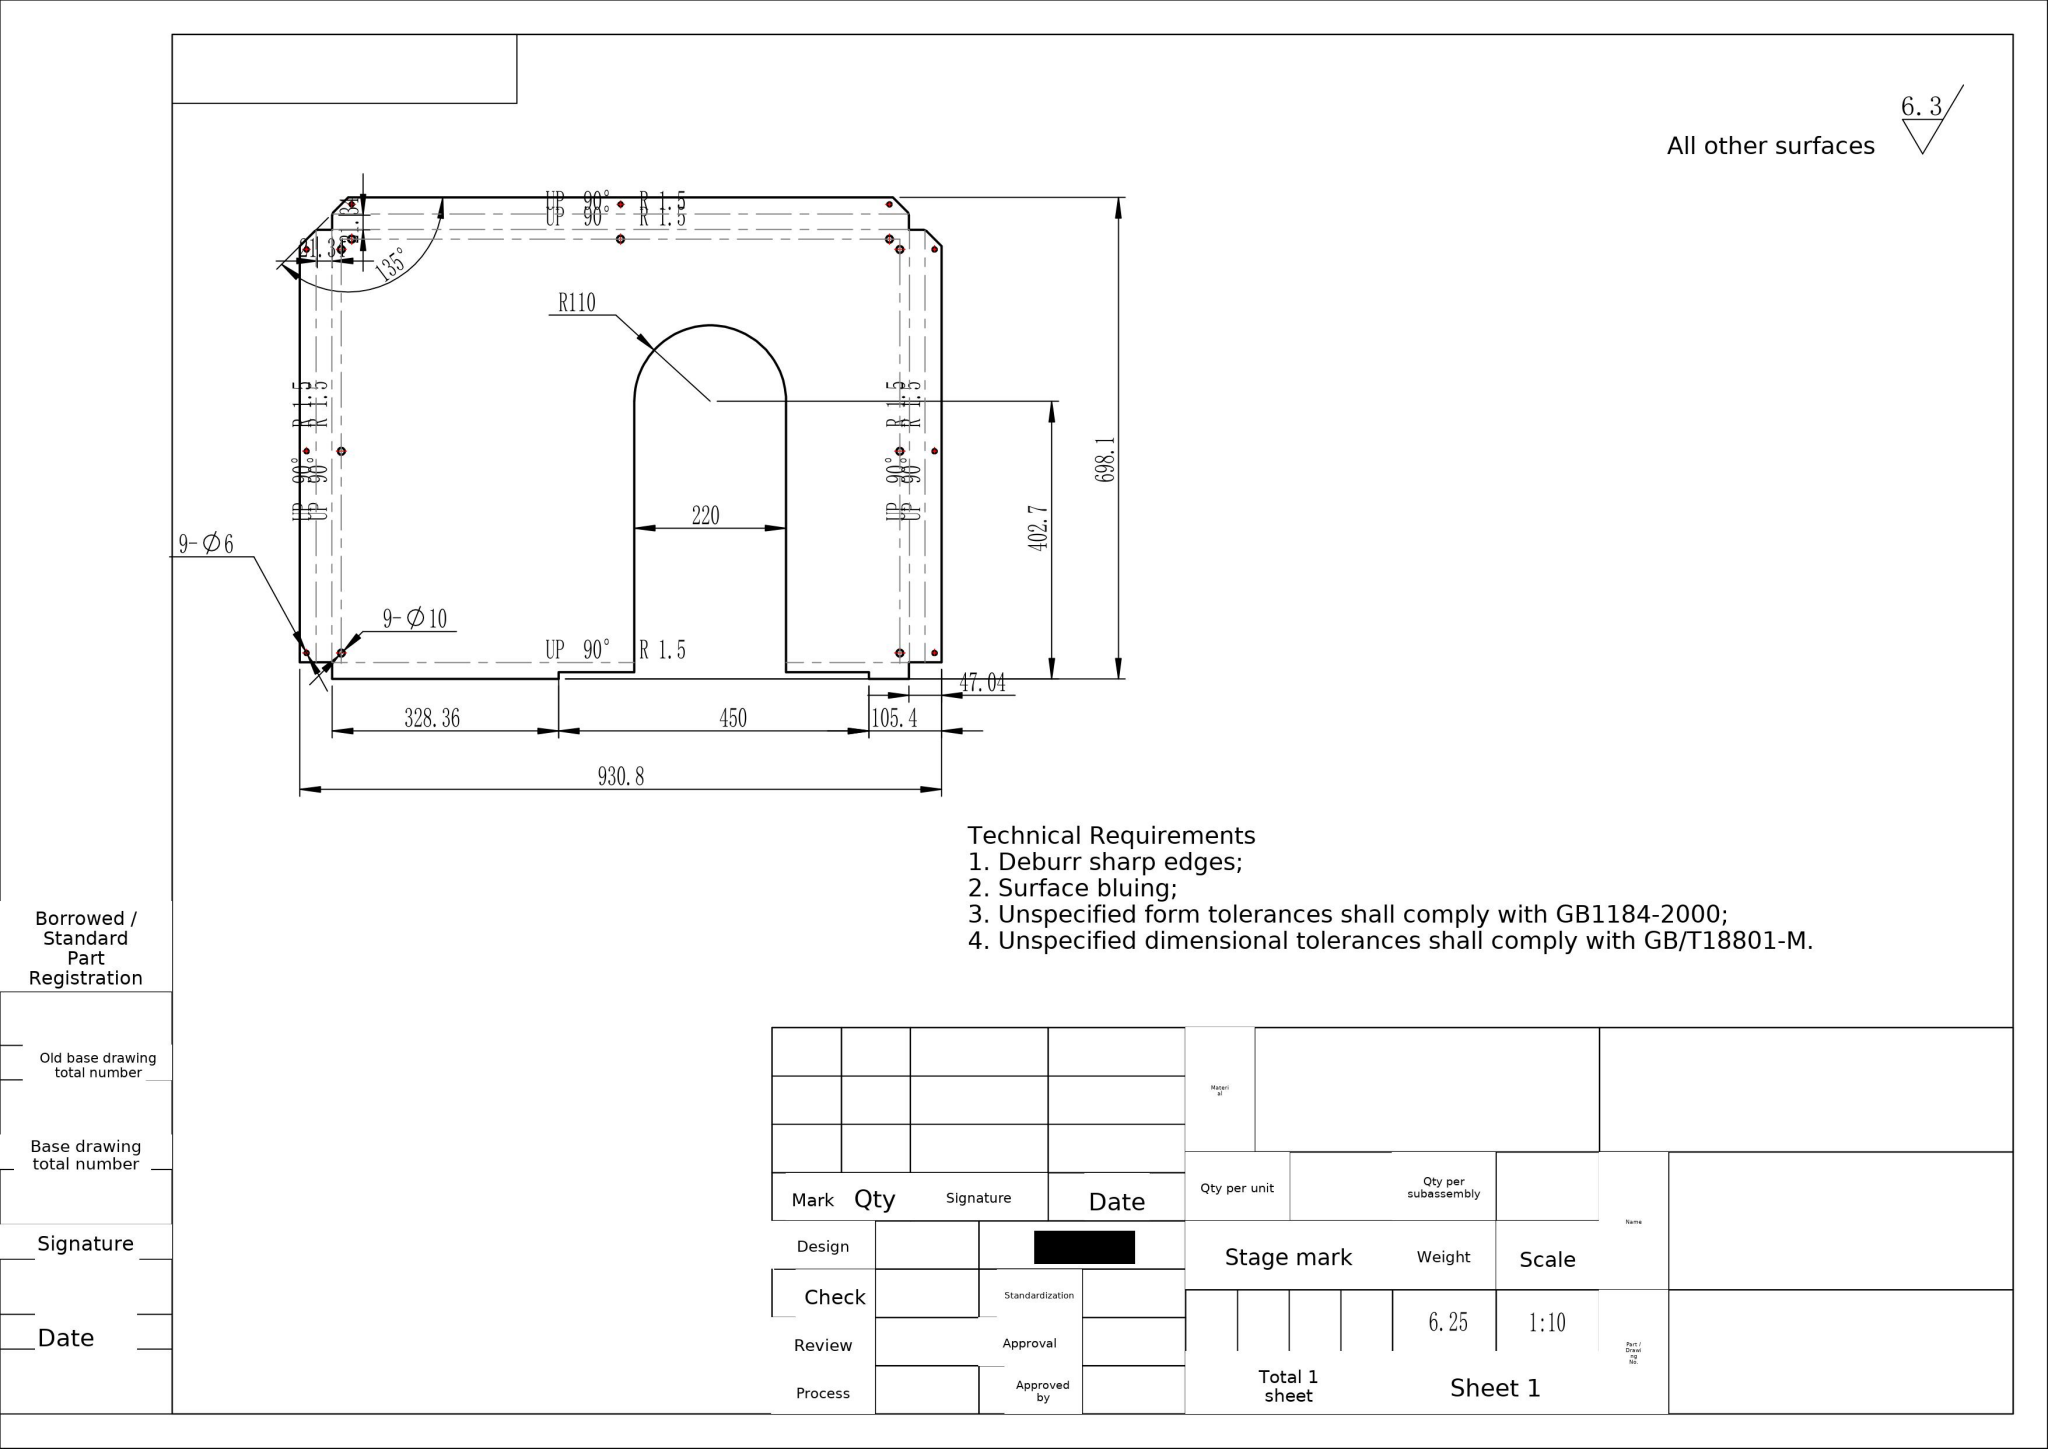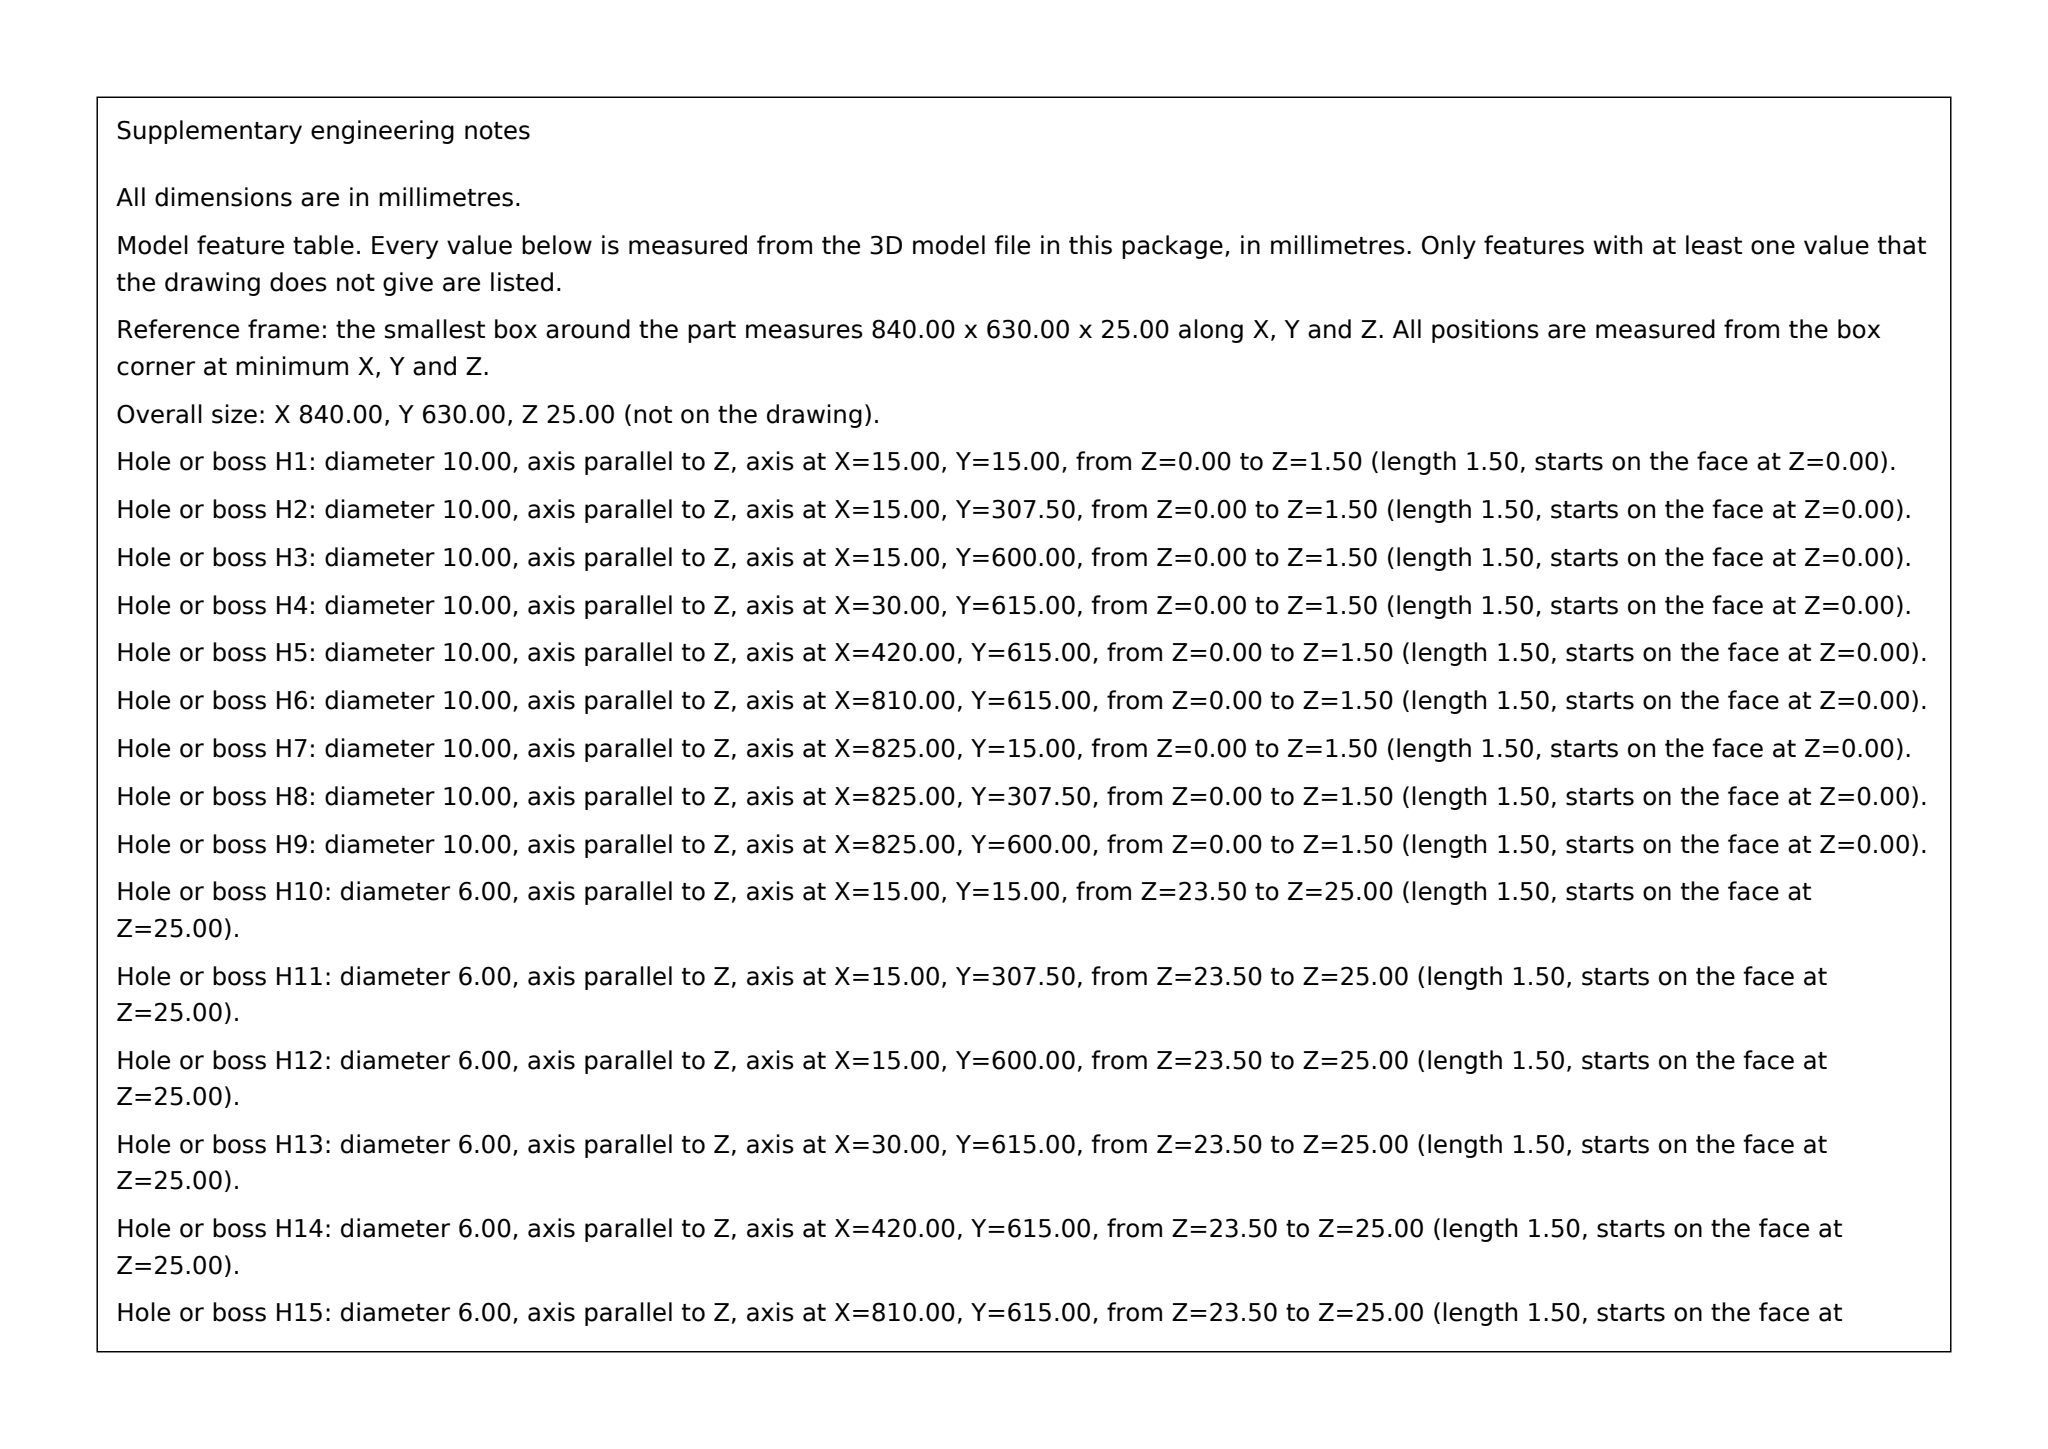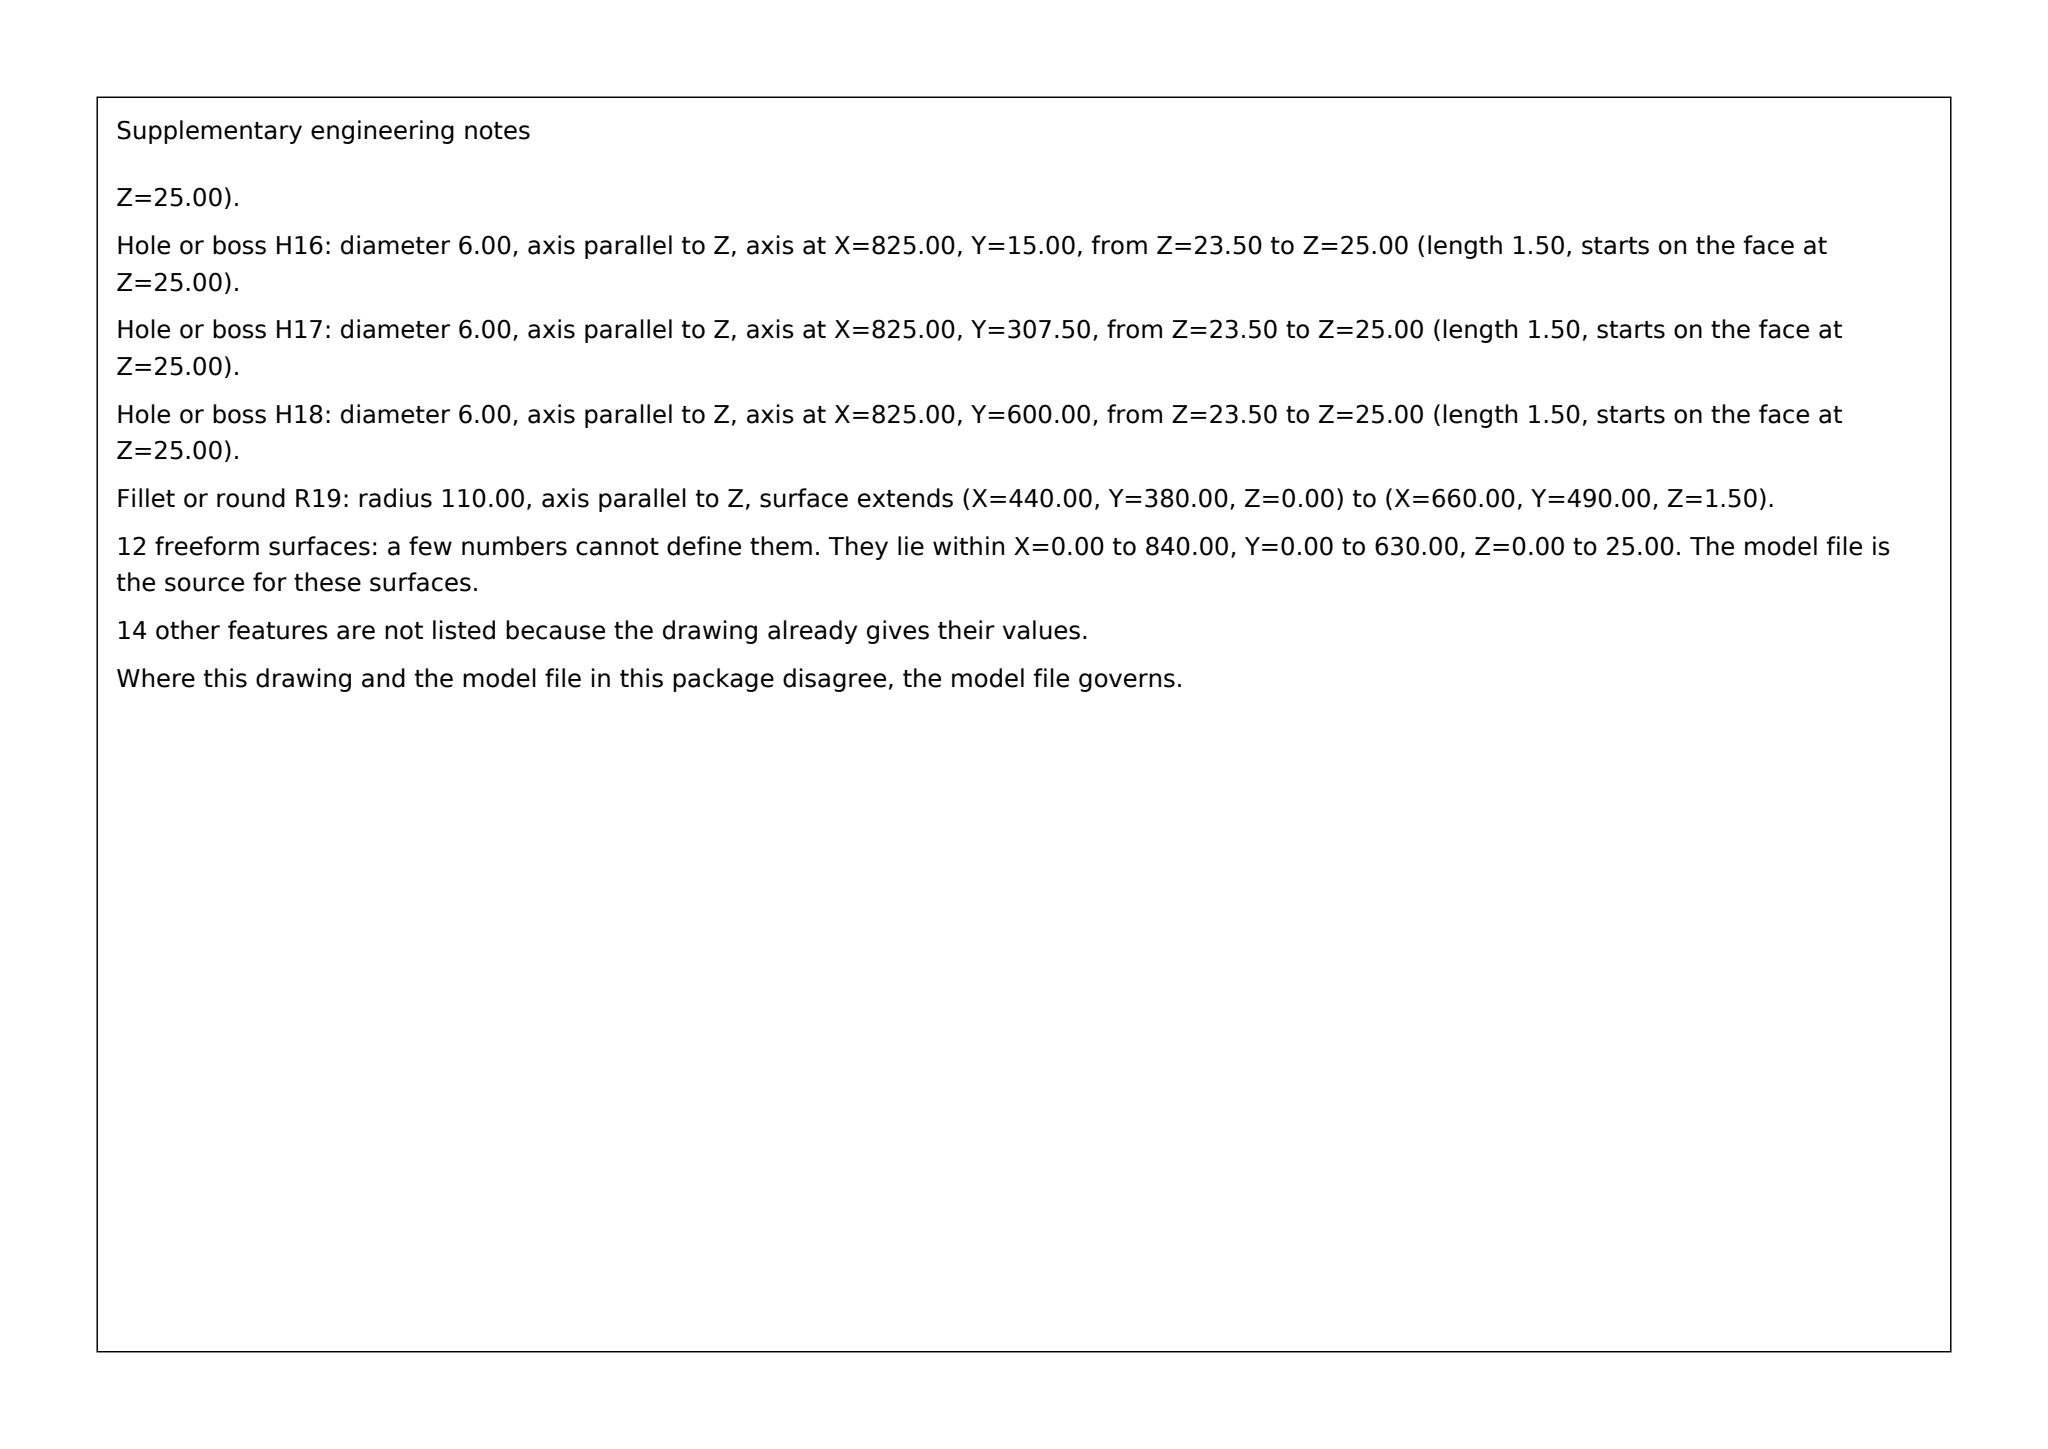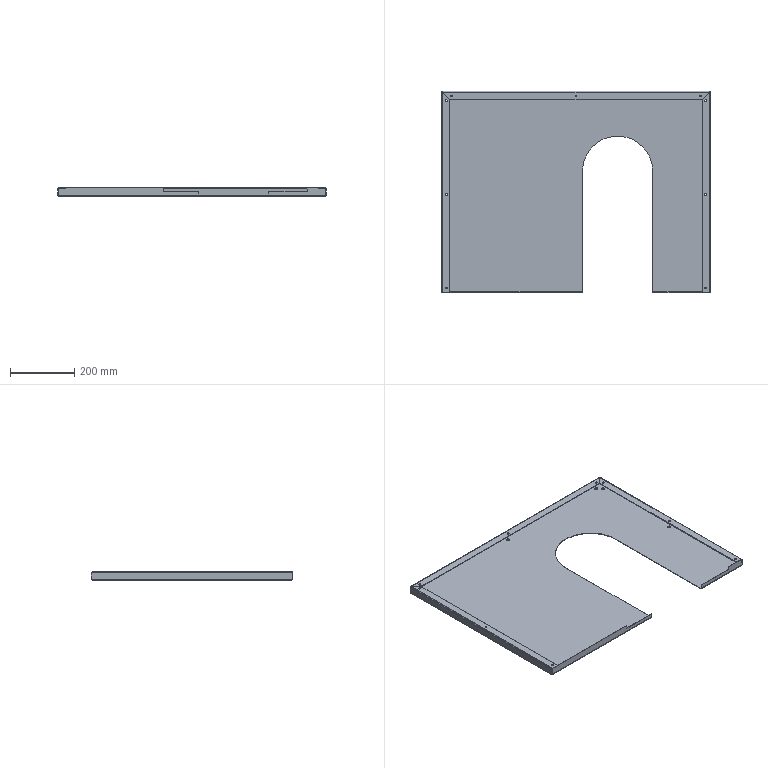Part | SolidWorks | mm | 1 solid | 114 faces | box 840 x 630 x 25 mm | volume 795444 mm3 | cylinder 53 | plane 49 | spline 12 | commonest cylinder face diameters 6 x26 10 x18 3 x8 220 x1